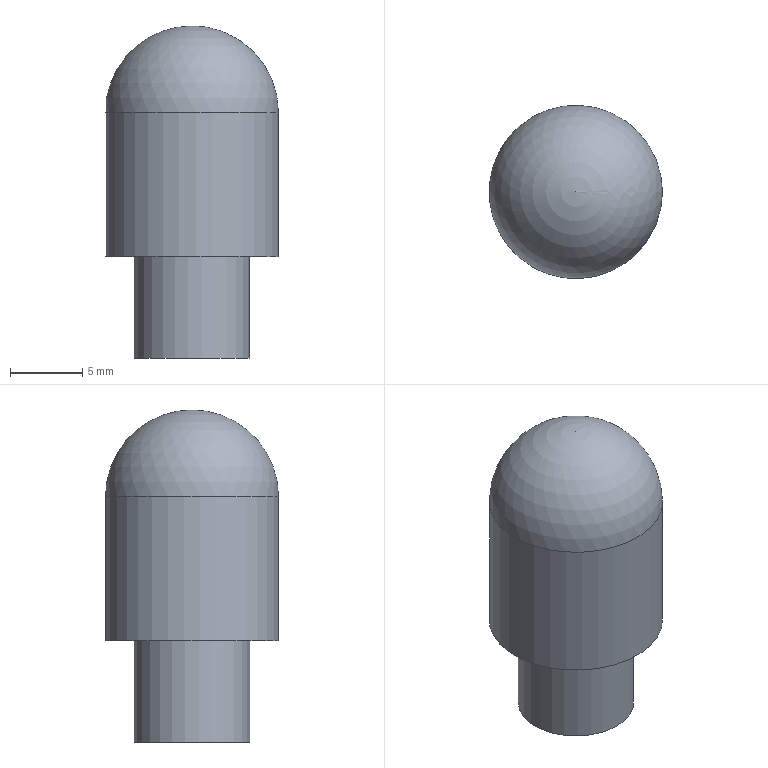Component | NX | 05B__27 | 1 solid | 7 faces | box 12 x 12 x 23 mm | volume 1811 mm3 | plane 3 | cylinder 3 | sphere 1 | commonest cylinder face diameters 8 x1 12 x1 4.2 x1
STEP:
#1=CARTESIAN_POINT('',(0.,0.,0.));
#2=DIRECTION('',(0.,0.,1.));
#3=DIRECTION('',(1.,0.,0.));
#4=AXIS2_PLACEMENT_3D('',#1,#2,#3);
#5=CARTESIAN_POINT('',(78.122,109.59,224.932));
#6=VERTEX_POINT('',#5);
#7=CARTESIAN_POINT('',(76.022,109.59,224.932));
#8=DIRECTION('',(0.,0.,1.));
#9=DIRECTION('',(1.,0.,0.));
#10=AXIS2_PLACEMENT_3D('',#7,#8,#9);
#11=CIRCLE('',#10,2.1);
#12=CARTESIAN_POINT('',(76.022,109.59,224.932));
#13=DIRECTION('',(0.,0.,1.));
#14=DIRECTION('',(1.,0.,0.));
#15=AXIS2_PLACEMENT_3D('',#12,#13,#14);
#16=PLANE('',#15);
#17=CARTESIAN_POINT('',(0.,0.));
#18=DIRECTION('',(1.,0.));
#19=AXIS2_PLACEMENT_2D('',#17,#18);
#20=CIRCLE('',#19,2.1);
#21=(GEOMETRIC_REPRESENTATION_CONTEXT(2)PARAMETRIC_REPRESENTATION_CONTEXT()REPRESENTATION_CONTEXT('',''));
#22=DEFINITIONAL_REPRESENTATION('',(#20),#21);
#23=PCURVE('',#16,#22);
#24=CARTESIAN_POINT('',(76.022,109.59,224.932));
#25=DIRECTION('',(0.,0.,1.));
#26=DIRECTION('',(1.,0.,0.));
#27=AXIS2_PLACEMENT_3D('',#24,#25,#26);
#28=CYLINDRICAL_SURFACE('',#27,2.1);
#29=CARTESIAN_POINT('',(0.,0.));
#30=DIRECTION('',(1.,0.));
#31=VECTOR('',#30,1.);
#32=LINE('',#29,#31);
#33=(GEOMETRIC_REPRESENTATION_CONTEXT(2)PARAMETRIC_REPRESENTATION_CONTEXT()REPRESENTATION_CONTEXT('',''));
#34=DEFINITIONAL_REPRESENTATION('',(#32),#33);
#35=PCURVE('',#28,#34);
#36=SURFACE_CURVE('',#11,(#23,#35),.PCURVE_S1.);
#37=EDGE_CURVE('',#6,#6,#36,.T.);
#38=ORIENTED_EDGE('',*,*,#37,.T.);
#39=EDGE_LOOP('',(#38));
#40=FACE_BOUND('',#39,.T.);
#41=CARTESIAN_POINT('',(80.022,109.59,224.932));
#42=VERTEX_POINT('',#41);
#43=CARTESIAN_POINT('',(76.022,109.59,224.932));
#44=DIRECTION('',(0.,0.,1.));
#45=DIRECTION('',(1.,0.,0.));
#46=AXIS2_PLACEMENT_3D('',#43,#44,#45);
#47=CIRCLE('',#46,4.);
#48=CARTESIAN_POINT('',(0.,0.));
#49=DIRECTION('',(1.,0.));
#50=AXIS2_PLACEMENT_2D('',#48,#49);
#51=CIRCLE('',#50,4.);
#52=(GEOMETRIC_REPRESENTATION_CONTEXT(2)PARAMETRIC_REPRESENTATION_CONTEXT()REPRESENTATION_CONTEXT('',''));
#53=DEFINITIONAL_REPRESENTATION('',(#51),#52);
#54=PCURVE('',#16,#53);
#55=CARTESIAN_POINT('',(76.022,109.59,224.932));
#56=DIRECTION('',(0.,0.,1.));
#57=DIRECTION('',(1.,0.,0.));
#58=AXIS2_PLACEMENT_3D('',#55,#56,#57);
#59=CYLINDRICAL_SURFACE('',#58,4.);
#60=CARTESIAN_POINT('',(0.,0.));
#61=DIRECTION('',(1.,0.));
#62=VECTOR('',#61,1.);
#63=LINE('',#60,#62);
#64=(GEOMETRIC_REPRESENTATION_CONTEXT(2)PARAMETRIC_REPRESENTATION_CONTEXT()REPRESENTATION_CONTEXT('',''));
#65=DEFINITIONAL_REPRESENTATION('',(#63),#64);
#66=PCURVE('',#59,#65);
#67=SURFACE_CURVE('',#47,(#54,#66),.PCURVE_S1.);
#68=EDGE_CURVE('',#42,#42,#67,.T.);
#69=ORIENTED_EDGE('',*,*,#68,.F.);
#70=EDGE_LOOP('',(#69));
#71=FACE_BOUND('',#70,.T.);
#72=ADVANCED_FACE('',(#40,#71),#16,.F.);
#73=CARTESIAN_POINT('',(80.022,109.59,231.932));
#74=VERTEX_POINT('',#73);
#75=CARTESIAN_POINT('',(76.022,109.59,231.932));
#76=DIRECTION('',(0.,0.,1.));
#77=DIRECTION('',(1.,0.,0.));
#78=AXIS2_PLACEMENT_3D('',#75,#76,#77);
#79=CIRCLE('',#78,4.);
#80=CARTESIAN_POINT('',(0.,7.));
#81=DIRECTION('',(1.,0.));
#82=VECTOR('',#81,1.);
#83=LINE('',#80,#82);
#84=(GEOMETRIC_REPRESENTATION_CONTEXT(2)PARAMETRIC_REPRESENTATION_CONTEXT()REPRESENTATION_CONTEXT('',''));
#85=DEFINITIONAL_REPRESENTATION('',(#83),#84);
#86=PCURVE('',#59,#85);
#87=CARTESIAN_POINT('',(80.022,109.59,231.932));
#88=DIRECTION('',(0.,0.,1.));
#89=DIRECTION('',(1.,0.,0.));
#90=AXIS2_PLACEMENT_3D('',#87,#88,#89);
#91=PLANE('',#90);
#92=CARTESIAN_POINT('',(-4.,0.));
#93=DIRECTION('',(1.,0.));
#94=AXIS2_PLACEMENT_2D('',#92,#93);
#95=CIRCLE('',#94,4.);
#96=(GEOMETRIC_REPRESENTATION_CONTEXT(2)PARAMETRIC_REPRESENTATION_CONTEXT()REPRESENTATION_CONTEXT('',''));
#97=DEFINITIONAL_REPRESENTATION('',(#95),#96);
#98=PCURVE('',#91,#97);
#99=SURFACE_CURVE('',#79,(#86,#98),.PCURVE_S1.);
#100=EDGE_CURVE('',#74,#74,#99,.T.);
#101=ORIENTED_EDGE('',*,*,#100,.F.);
#102=CARTESIAN_POINT('',(80.022,109.59,224.932));
#103=CARTESIAN_POINT('',(80.022,109.59,231.932));
#104=B_SPLINE_CURVE_WITH_KNOTS('',1,(#102,#103),.UNSPECIFIED.,.F.,.F.,(2,2),(0.,7.),.PIECEWISE_BEZIER_KNOTS.);
#105=CARTESIAN_POINT('',(0.,0.));
#106=DIRECTION('',(0.,1.));
#107=VECTOR('',#106,1.);
#108=LINE('',#105,#107);
#109=(GEOMETRIC_REPRESENTATION_CONTEXT(2)PARAMETRIC_REPRESENTATION_CONTEXT()REPRESENTATION_CONTEXT('',''));
#110=DEFINITIONAL_REPRESENTATION('',(#108),#109);
#111=PCURVE('',#59,#110);
#112=CARTESIAN_POINT('',(6.283,0.));
#113=DIRECTION('',(0.,1.));
#114=VECTOR('',#113,1.);
#115=LINE('',#112,#114);
#116=(GEOMETRIC_REPRESENTATION_CONTEXT(2)PARAMETRIC_REPRESENTATION_CONTEXT()REPRESENTATION_CONTEXT('',''));
#117=DEFINITIONAL_REPRESENTATION('',(#115),#116);
#118=PCURVE('',#59,#117);
#119=SEAM_CURVE('',#104,(#111,#118),.PCURVE_S1.);
#120=EDGE_CURVE('',#42,#74,#119,.T.);
#121=ORIENTED_EDGE('',*,*,#120,.F.);
#122=ORIENTED_EDGE('',*,*,#68,.T.);
#123=ORIENTED_EDGE('',*,*,#120,.T.);
#124=EDGE_LOOP('',(#101,#121,#122,#123));
#125=FACE_BOUND('',#124,.T.);
#126=ADVANCED_FACE('',(#125),#59,.T.);
#127=CARTESIAN_POINT('',(82.022,109.59,231.932));
#128=VERTEX_POINT('',#127);
#129=CARTESIAN_POINT('',(76.022,109.59,231.932));
#130=DIRECTION('',(0.,0.,1.));
#131=DIRECTION('',(1.,0.,0.));
#132=AXIS2_PLACEMENT_3D('',#129,#130,#131);
#133=CIRCLE('',#132,6.);
#134=CARTESIAN_POINT('',(-4.,0.));
#135=DIRECTION('',(1.,0.));
#136=AXIS2_PLACEMENT_2D('',#134,#135);
#137=CIRCLE('',#136,6.);
#138=(GEOMETRIC_REPRESENTATION_CONTEXT(2)PARAMETRIC_REPRESENTATION_CONTEXT()REPRESENTATION_CONTEXT('',''));
#139=DEFINITIONAL_REPRESENTATION('',(#137),#138);
#140=PCURVE('',#91,#139);
#141=CARTESIAN_POINT('',(76.022,109.59,224.932));
#142=DIRECTION('',(0.,0.,1.));
#143=DIRECTION('',(1.,0.,0.));
#144=AXIS2_PLACEMENT_3D('',#141,#142,#143);
#145=CYLINDRICAL_SURFACE('',#144,6.);
#146=CARTESIAN_POINT('',(0.,7.));
#147=DIRECTION('',(1.,0.));
#148=VECTOR('',#147,1.);
#149=LINE('',#146,#148);
#150=(GEOMETRIC_REPRESENTATION_CONTEXT(2)PARAMETRIC_REPRESENTATION_CONTEXT()REPRESENTATION_CONTEXT('',''));
#151=DEFINITIONAL_REPRESENTATION('',(#149),#150);
#152=PCURVE('',#145,#151);
#153=SURFACE_CURVE('',#133,(#140,#152),.PCURVE_S1.);
#154=EDGE_CURVE('',#128,#128,#153,.T.);
#155=ORIENTED_EDGE('',*,*,#154,.F.);
#156=EDGE_LOOP('',(#155));
#157=FACE_BOUND('',#156,.T.);
#158=ORIENTED_EDGE('',*,*,#100,.T.);
#159=EDGE_LOOP('',(#158));
#160=FACE_BOUND('',#159,.T.);
#161=ADVANCED_FACE('',(#157,#160),#91,.F.);
#162=CARTESIAN_POINT('',(82.022,109.59,241.932));
#163=VERTEX_POINT('',#162);
#164=CARTESIAN_POINT('',(76.022,109.59,241.932));
#165=DIRECTION('',(0.,0.,1.));
#166=DIRECTION('',(1.,0.,0.));
#167=AXIS2_PLACEMENT_3D('',#164,#165,#166);
#168=CIRCLE('',#167,6.);
#169=CARTESIAN_POINT('',(0.,17.));
#170=DIRECTION('',(1.,0.));
#171=VECTOR('',#170,1.);
#172=LINE('',#169,#171);
#173=(GEOMETRIC_REPRESENTATION_CONTEXT(2)PARAMETRIC_REPRESENTATION_CONTEXT()REPRESENTATION_CONTEXT('',''));
#174=DEFINITIONAL_REPRESENTATION('',(#172),#173);
#175=PCURVE('',#145,#174);
#176=CARTESIAN_POINT('',(76.022,109.59,241.932));
#177=DIRECTION('',(0.,0.,1.));
#178=DIRECTION('',(1.,0.,0.));
#179=AXIS2_PLACEMENT_3D('',#176,#177,#178);
#180=SPHERICAL_SURFACE('',#179,6.);
#181=CARTESIAN_POINT('',(0.,0.));
#182=CARTESIAN_POINT('',(0.0952,0.));
#183=CARTESIAN_POINT('',(0.2856,0.));
#184=CARTESIAN_POINT('',(0.5712,0.));
#185=CARTESIAN_POINT('',(0.8568,0.));
#186=CARTESIAN_POINT('',(1.142,0.));
#187=CARTESIAN_POINT('',(1.428,0.));
#188=CARTESIAN_POINT('',(1.714,0.));
#189=CARTESIAN_POINT('',(1.999,0.));
#190=CARTESIAN_POINT('',(2.285,0.));
#191=CARTESIAN_POINT('',(2.57,0.));
#192=CARTESIAN_POINT('',(2.856,0.));
#193=CARTESIAN_POINT('',(3.142,0.));
#194=CARTESIAN_POINT('',(3.427,0.));
#195=CARTESIAN_POINT('',(3.713,0.));
#196=CARTESIAN_POINT('',(3.998,0.));
#197=CARTESIAN_POINT('',(4.284,0.));
#198=CARTESIAN_POINT('',(4.57,0.));
#199=CARTESIAN_POINT('',(4.855,0.));
#200=CARTESIAN_POINT('',(5.141,0.));
#201=CARTESIAN_POINT('',(5.426,0.));
#202=CARTESIAN_POINT('',(5.712,0.));
#203=CARTESIAN_POINT('',(5.998,0.));
#204=CARTESIAN_POINT('',(6.188,0.));
#205=CARTESIAN_POINT('',(6.283,0.));
#206=B_SPLINE_CURVE_WITH_KNOTS('',3,(#181,#182,#183,#184,#185,#186,#187,#188,#189,#190,#191,#192,#193,#194,#195,#196,#197,#198,#199,#200,#201,#202,#203,#204,#205),.UNSPECIFIED.,.F.,.F.,(4,1,1,1,1,1,1,1,1,1,1,1,1,1,1,1,1,1,1,1,1,1,4),(0.,0.2856,0.5712,0.8568,1.142,1.428,1.714,1.999,2.285,2.57,2.856,3.142,3.427,3.713,3.998,4.284,4.57,4.855,5.141,5.426,5.712,5.998,6.283),.QUASI_UNIFORM_KNOTS.);
#207=(GEOMETRIC_REPRESENTATION_CONTEXT(2)PARAMETRIC_REPRESENTATION_CONTEXT()REPRESENTATION_CONTEXT('',''));
#208=DEFINITIONAL_REPRESENTATION('',(#206),#207);
#209=PCURVE('',#180,#208);
#210=SURFACE_CURVE('',#168,(#175,#209),.PCURVE_S1.);
#211=EDGE_CURVE('',#163,#163,#210,.T.);
#212=ORIENTED_EDGE('',*,*,#211,.F.);
#213=CARTESIAN_POINT('',(82.022,109.59,231.932));
#214=CARTESIAN_POINT('',(82.022,109.59,241.932));
#215=B_SPLINE_CURVE_WITH_KNOTS('',1,(#213,#214),.UNSPECIFIED.,.F.,.F.,(2,2),(7.,17.),.PIECEWISE_BEZIER_KNOTS.);
#216=CARTESIAN_POINT('',(0.,0.));
#217=DIRECTION('',(0.,1.));
#218=VECTOR('',#217,1.);
#219=LINE('',#216,#218);
#220=(GEOMETRIC_REPRESENTATION_CONTEXT(2)PARAMETRIC_REPRESENTATION_CONTEXT()REPRESENTATION_CONTEXT('',''));
#221=DEFINITIONAL_REPRESENTATION('',(#219),#220);
#222=PCURVE('',#145,#221);
#223=CARTESIAN_POINT('',(6.283,0.));
#224=DIRECTION('',(0.,1.));
#225=VECTOR('',#224,1.);
#226=LINE('',#223,#225);
#227=(GEOMETRIC_REPRESENTATION_CONTEXT(2)PARAMETRIC_REPRESENTATION_CONTEXT()REPRESENTATION_CONTEXT('',''));
#228=DEFINITIONAL_REPRESENTATION('',(#226),#227);
#229=PCURVE('',#145,#228);
#230=SEAM_CURVE('',#215,(#222,#229),.PCURVE_S1.);
#231=EDGE_CURVE('',#128,#163,#230,.T.);
#232=ORIENTED_EDGE('',*,*,#231,.F.);
#233=ORIENTED_EDGE('',*,*,#154,.T.);
#234=ORIENTED_EDGE('',*,*,#231,.T.);
#235=EDGE_LOOP('',(#212,#232,#233,#234));
#236=FACE_BOUND('',#235,.T.);
#237=ADVANCED_FACE('',(#236),#145,.T.);
#238=ORIENTED_EDGE('',*,*,#211,.T.);
#239=CARTESIAN_POINT('',(76.022,109.59,247.932));
#240=VERTEX_POINT('',#239);
#241=CARTESIAN_POINT('',(82.022,109.59,241.932));
#242=CARTESIAN_POINT('',(82.022,109.59,243.278));
#243=CARTESIAN_POINT('',(81.67,109.59,244.624));
#244=CARTESIAN_POINT('',(80.965,109.59,245.86));
#245=CARTESIAN_POINT('',(79.951,109.59,246.874));
#246=CARTESIAN_POINT('',(78.715,109.59,247.579));
#247=CARTESIAN_POINT('',(77.369,109.59,247.932));
#248=CARTESIAN_POINT('',(76.022,109.59,247.932));
#249=B_SPLINE_CURVE_WITH_KNOTS('',7,(#241,#242,#243,#244,#245,#246,#247,#248),.UNSPECIFIED.,.F.,.F.,(8,8),(0.,1.571),.PIECEWISE_BEZIER_KNOTS.);
#250=CARTESIAN_POINT('',(6.283,0.));
#251=DIRECTION('',(0.,1.));
#252=VECTOR('',#251,1.);
#253=LINE('',#250,#252);
#254=(GEOMETRIC_REPRESENTATION_CONTEXT(2)PARAMETRIC_REPRESENTATION_CONTEXT()REPRESENTATION_CONTEXT('',''));
#255=DEFINITIONAL_REPRESENTATION('',(#253),#254);
#256=PCURVE('',#180,#255);
#257=CARTESIAN_POINT('',(0.,0.));
#258=DIRECTION('',(0.,1.));
#259=VECTOR('',#258,1.);
#260=LINE('',#257,#259);
#261=(GEOMETRIC_REPRESENTATION_CONTEXT(2)PARAMETRIC_REPRESENTATION_CONTEXT()REPRESENTATION_CONTEXT('',''));
#262=DEFINITIONAL_REPRESENTATION('',(#260),#261);
#263=PCURVE('',#180,#262);
#264=SEAM_CURVE('',#249,(#256,#263),.PCURVE_S1.);
#265=EDGE_CURVE('',#163,#240,#264,.T.);
#266=ORIENTED_EDGE('',*,*,#265,.T.);
#267=ORIENTED_EDGE('',*,*,#265,.F.);
#268=EDGE_LOOP('',(#238,#266,#267));
#269=FACE_BOUND('',#268,.T.);
#270=ADVANCED_FACE('',(#269),#180,.T.);
#271=CARTESIAN_POINT('',(78.122,109.59,233.932));
#272=VERTEX_POINT('',#271);
#273=CARTESIAN_POINT('',(76.022,109.59,233.932));
#274=DIRECTION('',(0.,0.,1.));
#275=DIRECTION('',(1.,0.,0.));
#276=AXIS2_PLACEMENT_3D('',#273,#274,#275);
#277=CIRCLE('',#276,2.1);
#278=CARTESIAN_POINT('',(76.022,109.59,233.932));
#279=DIRECTION('',(0.,0.,1.));
#280=DIRECTION('',(1.,0.,0.));
#281=AXIS2_PLACEMENT_3D('',#278,#279,#280);
#282=PLANE('',#281);
#283=CARTESIAN_POINT('',(0.,0.));
#284=DIRECTION('',(1.,0.));
#285=AXIS2_PLACEMENT_2D('',#283,#284);
#286=CIRCLE('',#285,2.1);
#287=(GEOMETRIC_REPRESENTATION_CONTEXT(2)PARAMETRIC_REPRESENTATION_CONTEXT()REPRESENTATION_CONTEXT('',''));
#288=DEFINITIONAL_REPRESENTATION('',(#286),#287);
#289=PCURVE('',#282,#288);
#290=CARTESIAN_POINT('',(0.,9.));
#291=DIRECTION('',(1.,0.));
#292=VECTOR('',#291,1.);
#293=LINE('',#290,#292);
#294=(GEOMETRIC_REPRESENTATION_CONTEXT(2)PARAMETRIC_REPRESENTATION_CONTEXT()REPRESENTATION_CONTEXT('',''));
#295=DEFINITIONAL_REPRESENTATION('',(#293),#294);
#296=PCURVE('',#28,#295);
#297=SURFACE_CURVE('',#277,(#289,#296),.PCURVE_S1.);
#298=EDGE_CURVE('',#272,#272,#297,.T.);
#299=ORIENTED_EDGE('',*,*,#298,.F.);
#300=EDGE_LOOP('',(#299));
#301=FACE_BOUND('',#300,.T.);
#302=ADVANCED_FACE('',(#301),#282,.F.);
#303=ORIENTED_EDGE('',*,*,#298,.F.);
#304=CARTESIAN_POINT('',(78.122,109.59,224.932));
#305=CARTESIAN_POINT('',(78.122,109.59,233.932));
#306=B_SPLINE_CURVE_WITH_KNOTS('',1,(#304,#305),.UNSPECIFIED.,.F.,.F.,(2,2),(0.,9.),.PIECEWISE_BEZIER_KNOTS.);
#307=CARTESIAN_POINT('',(0.,0.));
#308=DIRECTION('',(0.,1.));
#309=VECTOR('',#308,1.);
#310=LINE('',#307,#309);
#311=(GEOMETRIC_REPRESENTATION_CONTEXT(2)PARAMETRIC_REPRESENTATION_CONTEXT()REPRESENTATION_CONTEXT('',''));
#312=DEFINITIONAL_REPRESENTATION('',(#310),#311);
#313=PCURVE('',#28,#312);
#314=CARTESIAN_POINT('',(6.283,0.));
#315=DIRECTION('',(0.,1.));
#316=VECTOR('',#315,1.);
#317=LINE('',#314,#316);
#318=(GEOMETRIC_REPRESENTATION_CONTEXT(2)PARAMETRIC_REPRESENTATION_CONTEXT()REPRESENTATION_CONTEXT('',''));
#319=DEFINITIONAL_REPRESENTATION('',(#317),#318);
#320=PCURVE('',#28,#319);
#321=SEAM_CURVE('',#306,(#313,#320),.PCURVE_S1.);
#322=EDGE_CURVE('',#6,#272,#321,.T.);
#323=ORIENTED_EDGE('',*,*,#322,.F.);
#324=ORIENTED_EDGE('',*,*,#37,.T.);
#325=ORIENTED_EDGE('',*,*,#322,.T.);
#326=EDGE_LOOP('',(#303,#323,#324,#325));
#327=FACE_BOUND('',#326,.F.);
#328=ADVANCED_FACE('',(#327),#28,.F.);
#329=CLOSED_SHELL('',(#72,#126,#161,#237,#270,#302,#328));
#330=MANIFOLD_SOLID_BREP('',#329);
#331=(LENGTH_UNIT()NAMED_UNIT(*)SI_UNIT(.MILLI.,.METRE.));
#332=UNCERTAINTY_MEASURE_WITH_UNIT(LENGTH_MEASURE(0.00001),#331,'','');
#333=(NAMED_UNIT(*)PLANE_ANGLE_UNIT()SI_UNIT($,.RADIAN.));
#334=(NAMED_UNIT(*)SI_UNIT($,.STERADIAN.)SOLID_ANGLE_UNIT());
#335=(GEOMETRIC_REPRESENTATION_CONTEXT(3)GLOBAL_UNCERTAINTY_ASSIGNED_CONTEXT((#332))GLOBAL_UNIT_ASSIGNED_CONTEXT((#331,#333,#334))REPRESENTATION_CONTEXT('',''));
#336=ADVANCED_BREP_SHAPE_REPRESENTATION('',(#4,#330),#335);